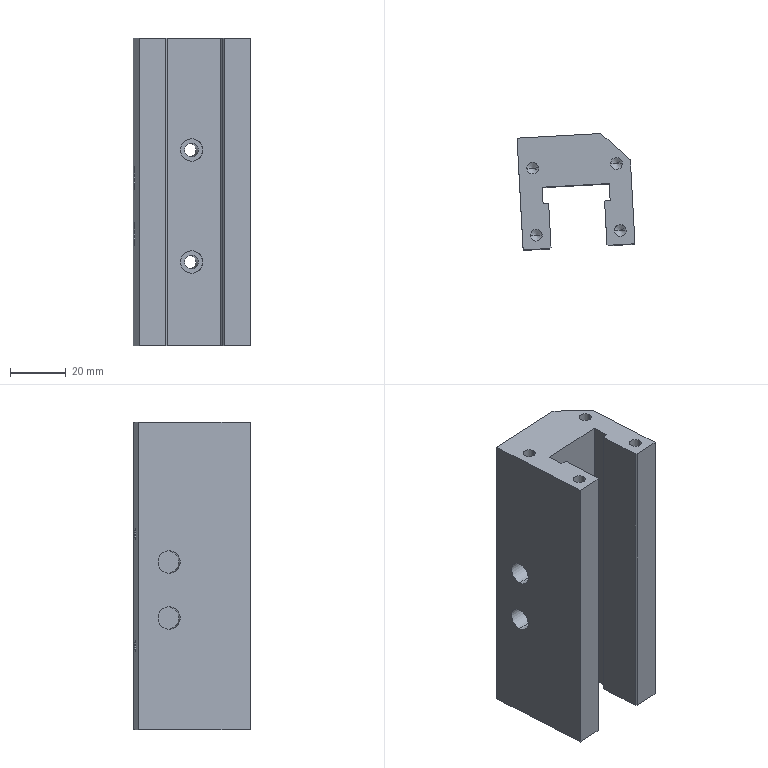Component | SolidWorks | T160418-M01U03-P04A-1 | 1 solid | 67 faces | box 42.13 x 41.58 x 110 mm | volume 116056 mm3 | cylinder 28 | plane 23 | cone 16 | commonest cylinder face diameters 4.2 x16 8 x8 5 x4 | material Tin Bronze
build123d program:
from build123d import *

# Parameters (mm, degrees)
SKETCH1_W                    = 110
SKETCH1_H                    = 40
BOSS_EXTRUDE1_DEPTH          = 20
CUT_EXTRUDE3_DEPTH           = 114.578
M5_TAPPED_HOLE1_D            = 4.2
M5_TAPPED_HOLE1_DEPTH        = 14
M5_TAPPED_HOLE1_TIP          = 1.262
CHAMFER2_SIZE                = 10
CHAMFER3_SIZE                = 0.2
CHAMFER4_SIZE                = 0.5
M6_TAPPED_HOLE1_D            = 5
SKETCH17_R                   = 4
CUT_EXTRUDE5_DEPTH           = 1
M5_TAPPED_HOLE2_D            = 4.2
M5_TAPPED_HOLE2_DEPTH        = 14
M5_TAPPED_HOLE2_TIP          = 1.262
F_8_0_8_DIAMETER_HOLE2_D     = 8
F_8_0_8_DIAMETER_HOLE2_DEPTH = 10


with BuildPart() as part:
    # Sketch1 → Boss-Extrude1 (new, symmetric)
    with BuildSketch(Plane.XY):
        Rectangle(SKETCH1_W, SKETCH1_H)
    extrude(amount=BOSS_EXTRUDE1_DEPTH, both=True)

    # Sketch5 → Cut-Extrude3 (cut, through all)
    with BuildSketch(Plane(origin=(55, 0, 0), x_dir=(0, 0, -1), z_dir=(1, 0, 0))):
        Polygon((-10, 20), (-10, 4), (-12, 4), (-12, -2), (12, -2), (12, 4), (10, 4), (10, 20), align=None)
    extrude(amount=-CUT_EXTRUDE3_DEPTH, mode=Mode.SUBTRACT)

    # M5 Tapped Hole1
    with Locations(Plane(origin=(-55, -18.814, 2.59), x_dir=(0, 0, -1), z_dir=(-1, 0, 0))):
        with Locations((-12.41, -33.814), (-12.41, -9.814), (17.59, -9.814), (17.59, -33.814)):
            Hole(M5_TAPPED_HOLE1_D / 2, depth=M5_TAPPED_HOLE1_DEPTH)
            with Locations((0, 0, -(M5_TAPPED_HOLE1_DEPTH + M5_TAPPED_HOLE1_TIP / 2))):  # 118° drill point
                Cone(0, M5_TAPPED_HOLE1_D / 2, M5_TAPPED_HOLE1_TIP, mode=Mode.SUBTRACT)

    # Chamfer2
    chamfer2_edges = [part.edges().sort_by_distance(p)[0] for p in [
        (0, -20, -20),
    ]]
    chamfer(chamfer2_edges, length=CHAMFER2_SIZE)

    # Chamfer3
    chamfer3_edges = [part.edges().sort_by_distance(p)[0] for p in [
        (0, 4, -10),
        (0, 4, 10),
    ]]
    chamfer(chamfer3_edges, length=CHAMFER3_SIZE)

    # Chamfer4
    chamfer4_edges = [part.edges().sort_by_distance(p)[0] for p in [
        (0, 20, 10),
        (0, 20, -10),
    ]]
    chamfer(chamfer4_edges, length=CHAMFER4_SIZE)

    # M6 Tapped Hole1 (through all)
    with Locations(Plane.XZ.offset(20)):
        with Locations((-15, 0), (25, 0)):
            Hole(M6_TAPPED_HOLE1_D / 2)

    # Sketch17 → Cut-Extrude5 (cut)
    with BuildSketch(Plane(origin=(0, -2, 0), x_dir=(1, 0, 0), z_dir=(0, 1, 0))):
        with Locations(Location((-15, 0, 0), (0, 0, 180))):
            Circle(SKETCH17_R)
        with Locations(Location((25, 0, 0), (0, 0, 180))):
            Circle(SKETCH17_R)
    extrude(amount=-CUT_EXTRUDE5_DEPTH, mode=Mode.SUBTRACT)

    # M5 Tapped Hole2
    with Locations(Plane(origin=(55, 0, 0), x_dir=(0, 0, -1), z_dir=(1, 0, 0))):
        with Locations((-15, -9), (5, -9), (15, 15), (-15, 15)):
            Hole(M5_TAPPED_HOLE2_D / 2, depth=M5_TAPPED_HOLE2_DEPTH)
            with Locations((0, 0, -(M5_TAPPED_HOLE2_DEPTH + M5_TAPPED_HOLE2_TIP / 2))):  # 118° drill point
                Cone(0, M5_TAPPED_HOLE2_D / 2, M5_TAPPED_HOLE2_TIP, mode=Mode.SUBTRACT)

    # 8.0 _8_ Diameter Hole2
    with Locations(Plane.XY.offset(20)):
        with Locations((15, -9), (-5, -9)):
            Hole(F_8_0_8_DIAMETER_HOLE2_D / 2, depth=F_8_0_8_DIAMETER_HOLE2_DEPTH)


solid = part.part

# Placed as in the assembly
solid = solid.moved(Location((511.102, 149.336, -223.818), (90, -86.863, -90)))